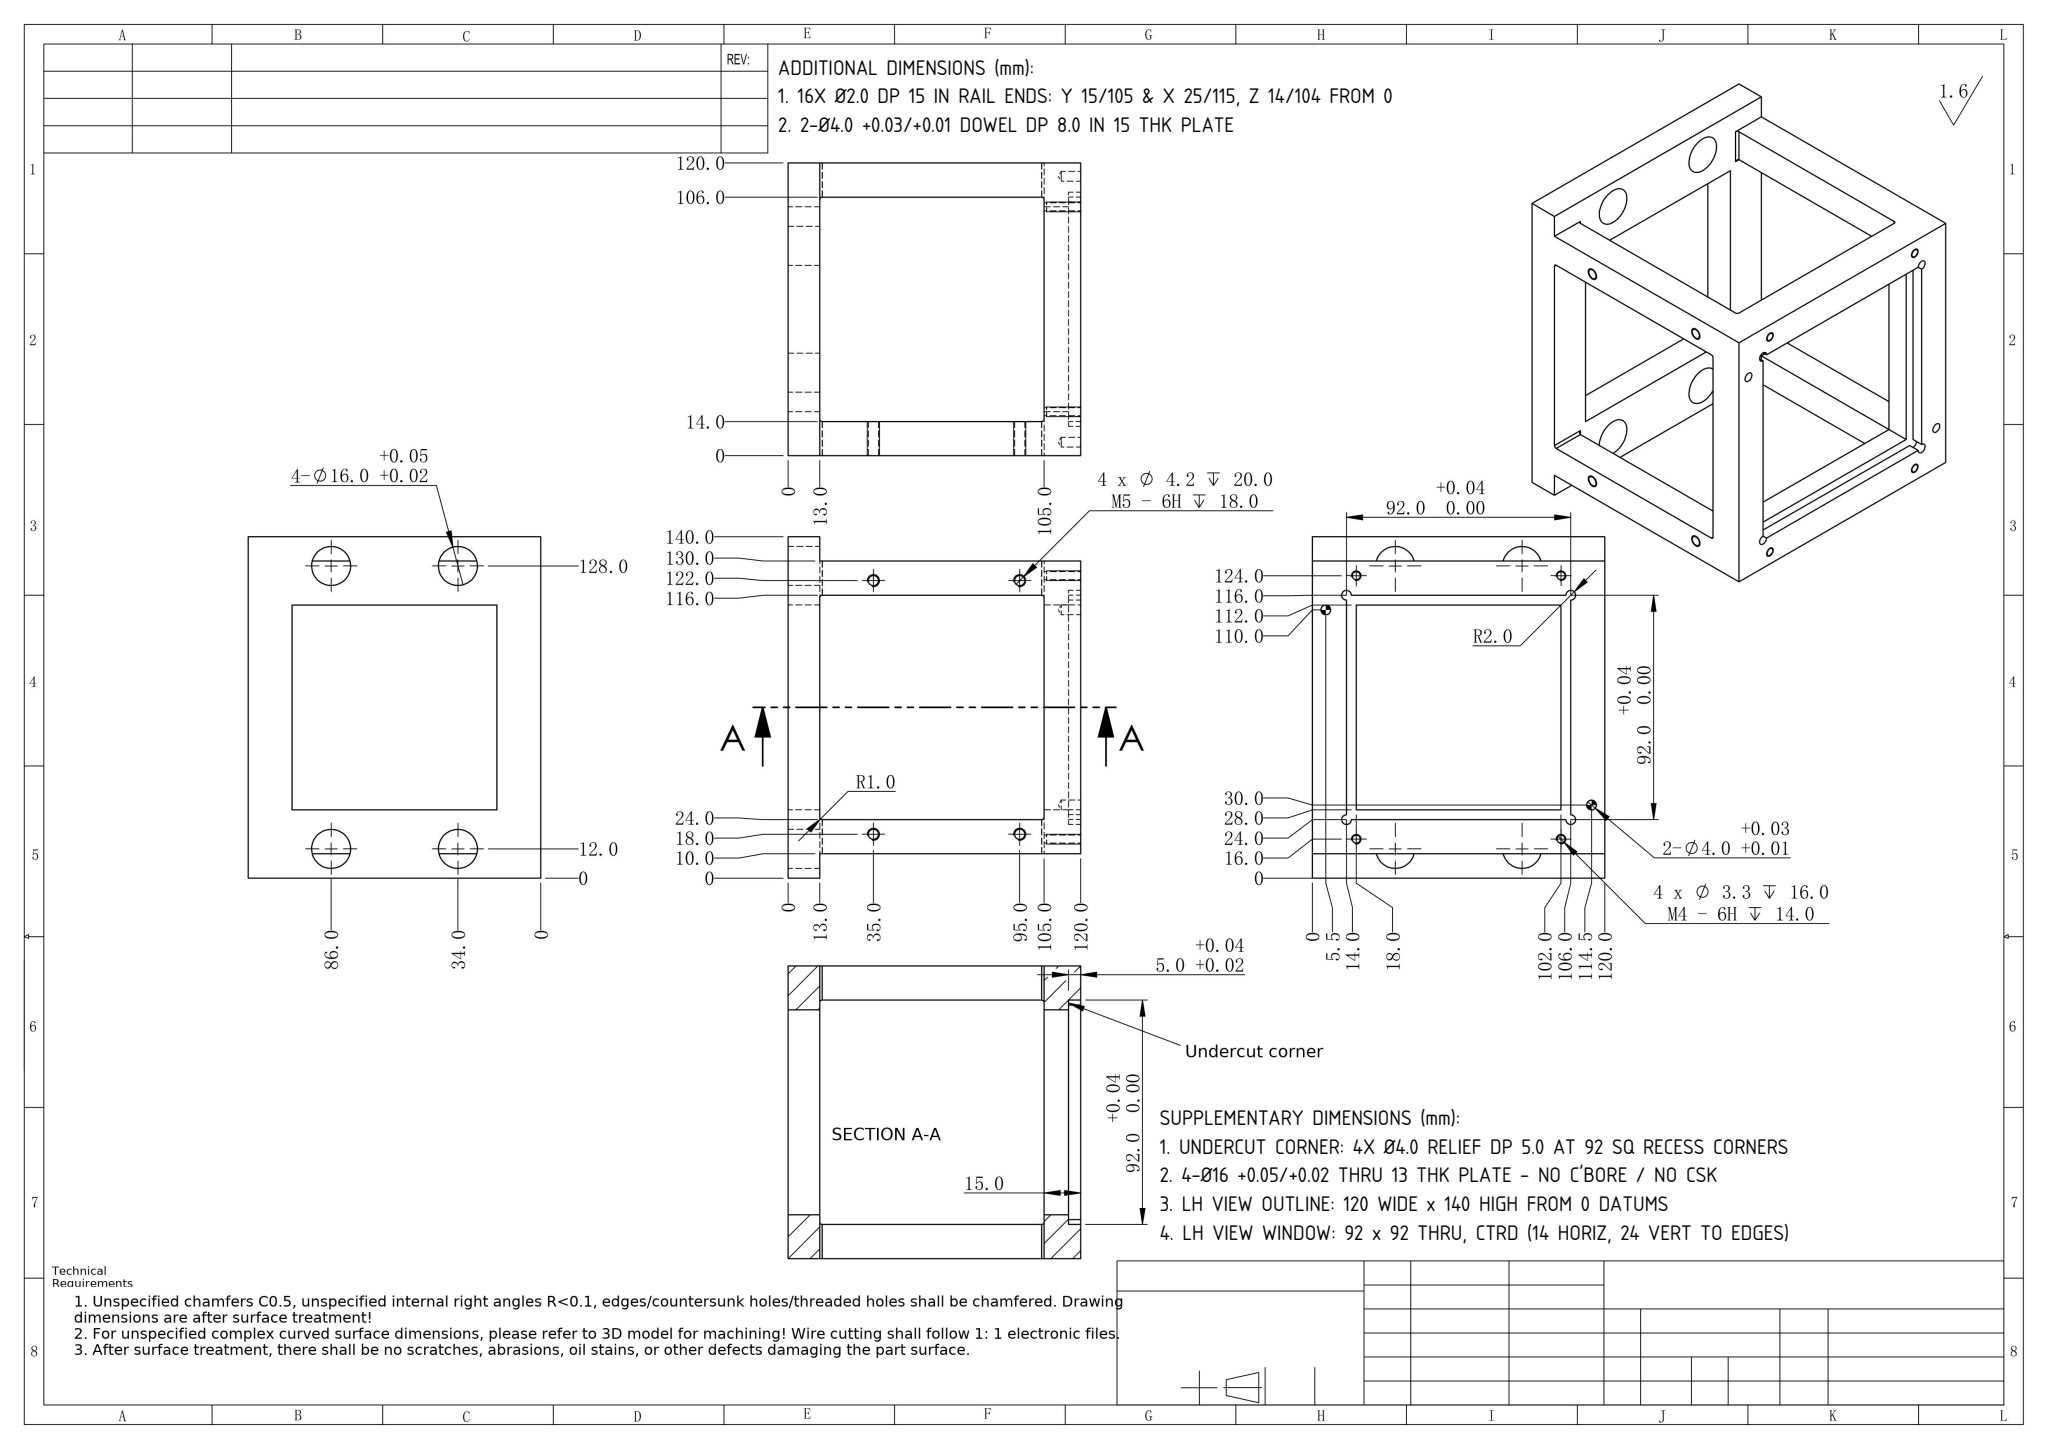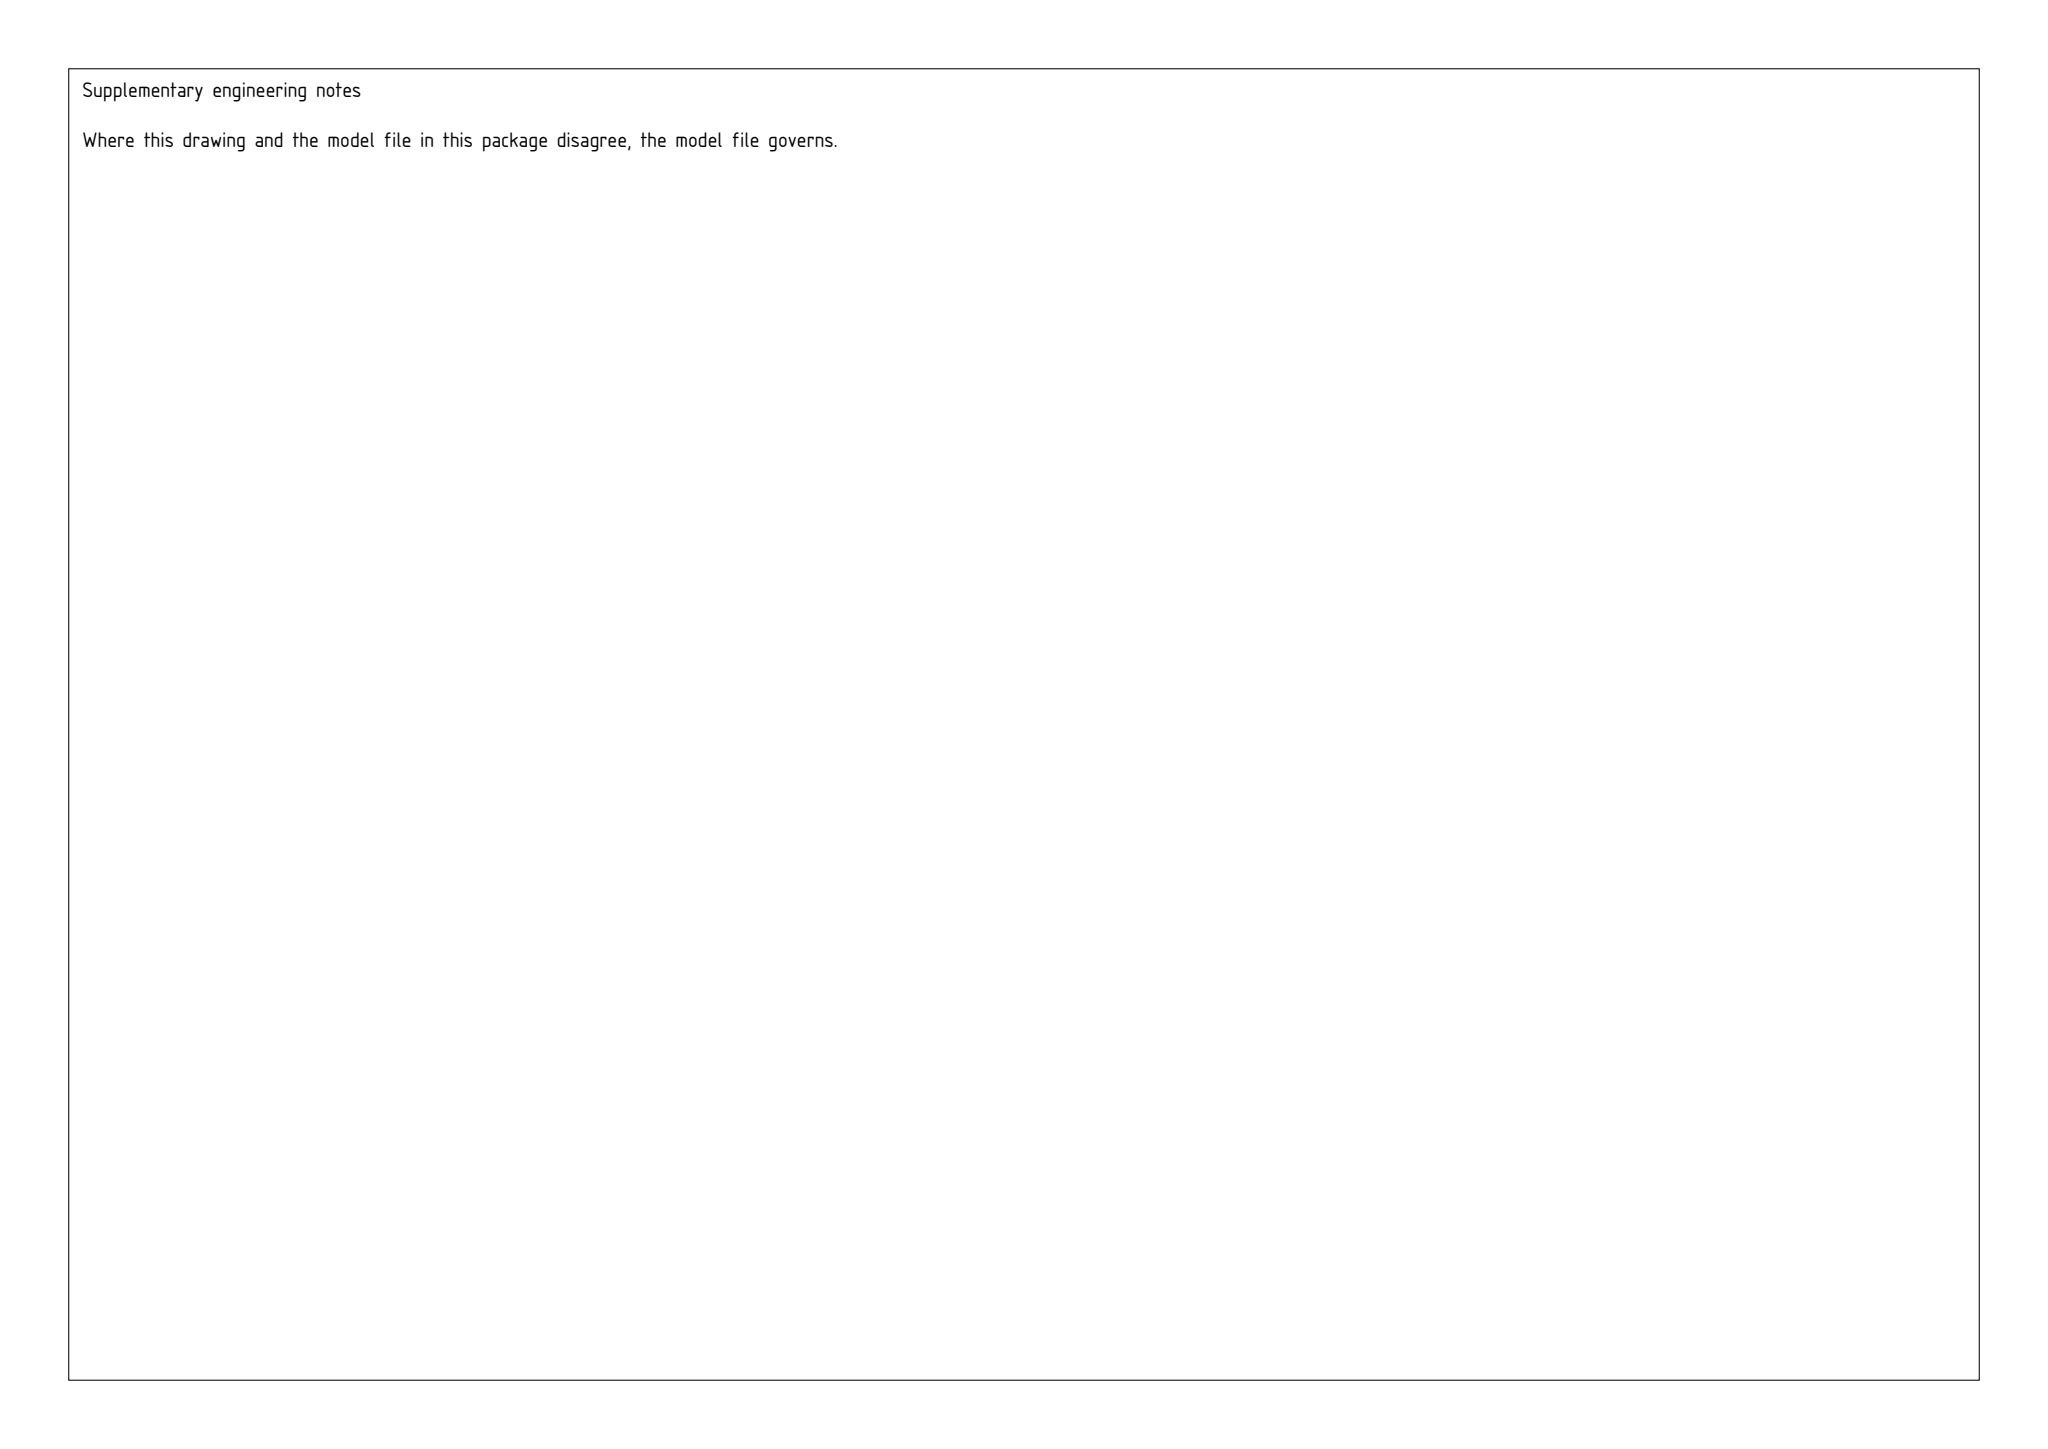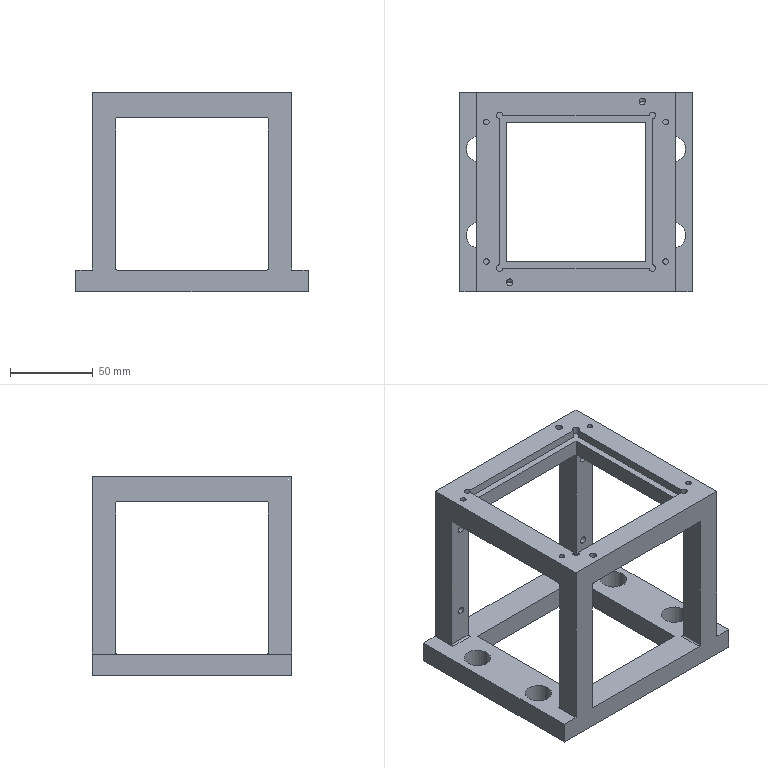Part | SolidWorks | mm | 1 solid | 85 faces | box 140 x 120 x 120 mm | volume 289825 mm3 | cylinder 50 | plane 31 | cone 4 | commonest cylinder face diameters 2 x16 4 x10 4.2 x8 16 x8 3.3 x8
build123d program:
from build123d import *

# Parameters (mm, degrees)
SKETCH1_W                      = 120
SKETCH1_H                      = 120
BOSS_EXTRUDE1_DEPTH            = 60
SKETCH5_W                      = 84
SKETCH5_H                      = 84
CUT_EXTRUDE3_DEPTH             = 147.969
SKETCH6_W                      = 92
SKETCH6_H                      = 92
CUT_EXTRUDE4_DEPTH             = 5
M4_TAPPED_HOLE1_D              = 3.3
M4_TAPPED_HOLE1_DEPTH          = 16
M4_TAPPED_HOLE1_TIP            = 0.9914
SIZE_MM_DOWEL_PIN_HOLE_1_D     = 4
SIZE_MM_DOWEL_PIN_HOLE_1_DEPTH = 8
SIZE_MM_DOWEL_PIN_HOLE_1_TIP   = 1.202
SKETCH11_R                     = 2
CUT_EXTRUDE5_DEPTH             = 5
CUT_EXTRUDE6_DEPTH             = 147.969
CUT_EXTRUDE7_DEPTH             = 147.969
SKETCH15_W                     = 13
SKETCH15_H                     = 120
BOSS_EXTRUDE3_DEPTH            = 10
SKETCH16_W                     = 13
SKETCH16_H                     = 120
BOSS_EXTRUDE4_DEPTH            = 10
SKETCH17_R                     = 8
CUT_EXTRUDE8_DEPTH             = 15
M5_TAPPED_HOLE1_D              = 4.2
M5_TAPPED_HOLE1_DEPTH          = 20
M5_TAPPED_HOLE1_TIP            = 1.262


with BuildPart() as part:
    # Sketch1 → Boss-Extrude1 (new, symmetric)
    with BuildSketch(Plane.XY):
        Rectangle(SKETCH1_W, SKETCH1_H)
    extrude(amount=BOSS_EXTRUDE1_DEPTH, both=True)

    # Sketch5 → Cut-Extrude3 (cut, through all)
    with BuildSketch(Plane.XY.offset(60)):
        Rectangle(SKETCH5_W, SKETCH5_H)
    extrude(amount=-CUT_EXTRUDE3_DEPTH, mode=Mode.SUBTRACT)

    # Sketch6 → Cut-Extrude4 (cut)
    with BuildSketch(Plane.XY.offset(60)):
        Rectangle(SKETCH6_W, SKETCH6_H)
    extrude(amount=-CUT_EXTRUDE4_DEPTH, mode=Mode.SUBTRACT)

    # M4 Tapped Hole1
    with Locations(Plane.XY.offset(60)):
        with Locations((54, 42), (54, -42), (-54, 42), (-54, -42)):
            Hole(M4_TAPPED_HOLE1_D / 2, depth=M4_TAPPED_HOLE1_DEPTH)
            with Locations((0, 0, -(M4_TAPPED_HOLE1_DEPTH + M4_TAPPED_HOLE1_TIP / 2))):  # 118° drill point
                Cone(0, M4_TAPPED_HOLE1_D / 2, M4_TAPPED_HOLE1_TIP, mode=Mode.SUBTRACT)

    # Size mm Dowel Pin Hole 1
    with Locations(Plane.XY.offset(60)):
        with Locations((40, 54.5), (-40, -54.5)):
            Hole(SIZE_MM_DOWEL_PIN_HOLE_1_D / 2, depth=SIZE_MM_DOWEL_PIN_HOLE_1_DEPTH)
            with Locations((0, 0, -(SIZE_MM_DOWEL_PIN_HOLE_1_DEPTH + SIZE_MM_DOWEL_PIN_HOLE_1_TIP / 2))):  # 118° drill point
                Cone(0, SIZE_MM_DOWEL_PIN_HOLE_1_D / 2, SIZE_MM_DOWEL_PIN_HOLE_1_TIP, mode=Mode.SUBTRACT)

    # Sketch11 → Cut-Extrude5 (cut)
    with BuildSketch(Plane.XY.offset(60)):
        with Locations((-46, 46)):
            Circle(SKETCH11_R)
        with Locations((46, 46)):
            Circle(SKETCH11_R)
        with Locations((-46, -46)):
            Circle(SKETCH11_R)
        with Locations((46, -46)):
            Circle(SKETCH11_R)
    extrude(amount=-CUT_EXTRUDE5_DEPTH, mode=Mode.SUBTRACT)

    # Sketch12 → Cut-Extrude6 (cut, through all)
    with BuildSketch(Plane.XZ.offset(60)):
        with BuildLine():
            Line((-45, 45), (45, 45))
            ThreePointArc((45, 45), (45.707, 44.707), (46, 44))
            Line((46, 44), (46, -46))
            ThreePointArc((46, -46), (45.707, -46.707), (45, -47))
            Line((45, -47), (-45, -47))
            ThreePointArc((-45, -47), (-45.707, -46.707), (-46, -46))
            Line((-46, -46), (-46, 44))
            ThreePointArc((-46, 44), (-45.707, 44.707), (-45, 45))
        make_face()
    extrude(amount=-CUT_EXTRUDE6_DEPTH, mode=Mode.SUBTRACT)

    # Sketch13 → Cut-Extrude7 (cut, through all)
    with BuildSketch(Plane.ZY.offset(60)):
        with BuildLine():
            Line((44, 46), (-46, 46))
            ThreePointArc((-46, 46), (-46.707, 45.707), (-47, 45))
            Line((-47, 45), (-47, -45))
            ThreePointArc((-47, -45), (-46.707, -45.707), (-46, -46))
            Line((-46, -46), (44, -46))
            ThreePointArc((44, -46), (44.707, -45.707), (45, -45))
            Line((45, -45), (45, 45))
            ThreePointArc((45, 45), (44.707, 45.707), (44, 46))
        make_face()
    extrude(amount=-CUT_EXTRUDE7_DEPTH, mode=Mode.SUBTRACT)

    # Sketch15 → Boss-Extrude3 (add)
    with BuildSketch(Plane.ZY.offset(60)):
        with Locations((-53.5, 0)):
            Rectangle(SKETCH15_W, SKETCH15_H)
    extrude(amount=BOSS_EXTRUDE3_DEPTH)

    # Sketch16 → Boss-Extrude4 (add)
    with BuildSketch(Plane(origin=(60, 0, 0), x_dir=(0, 0, -1), z_dir=(1, 0, 0))):
        with Locations((53.5, 0)):
            Rectangle(SKETCH16_W, SKETCH16_H)
    extrude(amount=BOSS_EXTRUDE4_DEPTH)

    # Sketch17 → Cut-Extrude8 (cut)
    with BuildSketch(Plane(origin=(0, 0, -60), x_dir=(-1, 0, 0), z_dir=(0, 0, -1))):
        with Locations((-58, 26)):
            Circle(SKETCH17_R)
        with Locations((-58, -26)):
            Circle(SKETCH17_R)
        with Locations((58, 26)):
            Circle(SKETCH17_R)
        with Locations((58, -26)):
            Circle(SKETCH17_R)
    extrude(amount=-CUT_EXTRUDE8_DEPTH, mode=Mode.SUBTRACT)

    # M5 Tapped Hole1
    with Locations(Plane(origin=(0, 60, 0), x_dir=(1, 0, 0), z_dir=(0, 1, 0))):
        with Locations((52, -35), (52, 25), (-52, -35), (-52, 25)):
            Hole(M5_TAPPED_HOLE1_D / 2, depth=M5_TAPPED_HOLE1_DEPTH)
            with Locations((0, 0, -(M5_TAPPED_HOLE1_DEPTH + M5_TAPPED_HOLE1_TIP / 2))):  # 118° drill point
                Cone(0, M5_TAPPED_HOLE1_D / 2, M5_TAPPED_HOLE1_TIP, mode=Mode.SUBTRACT)


solid = part.part